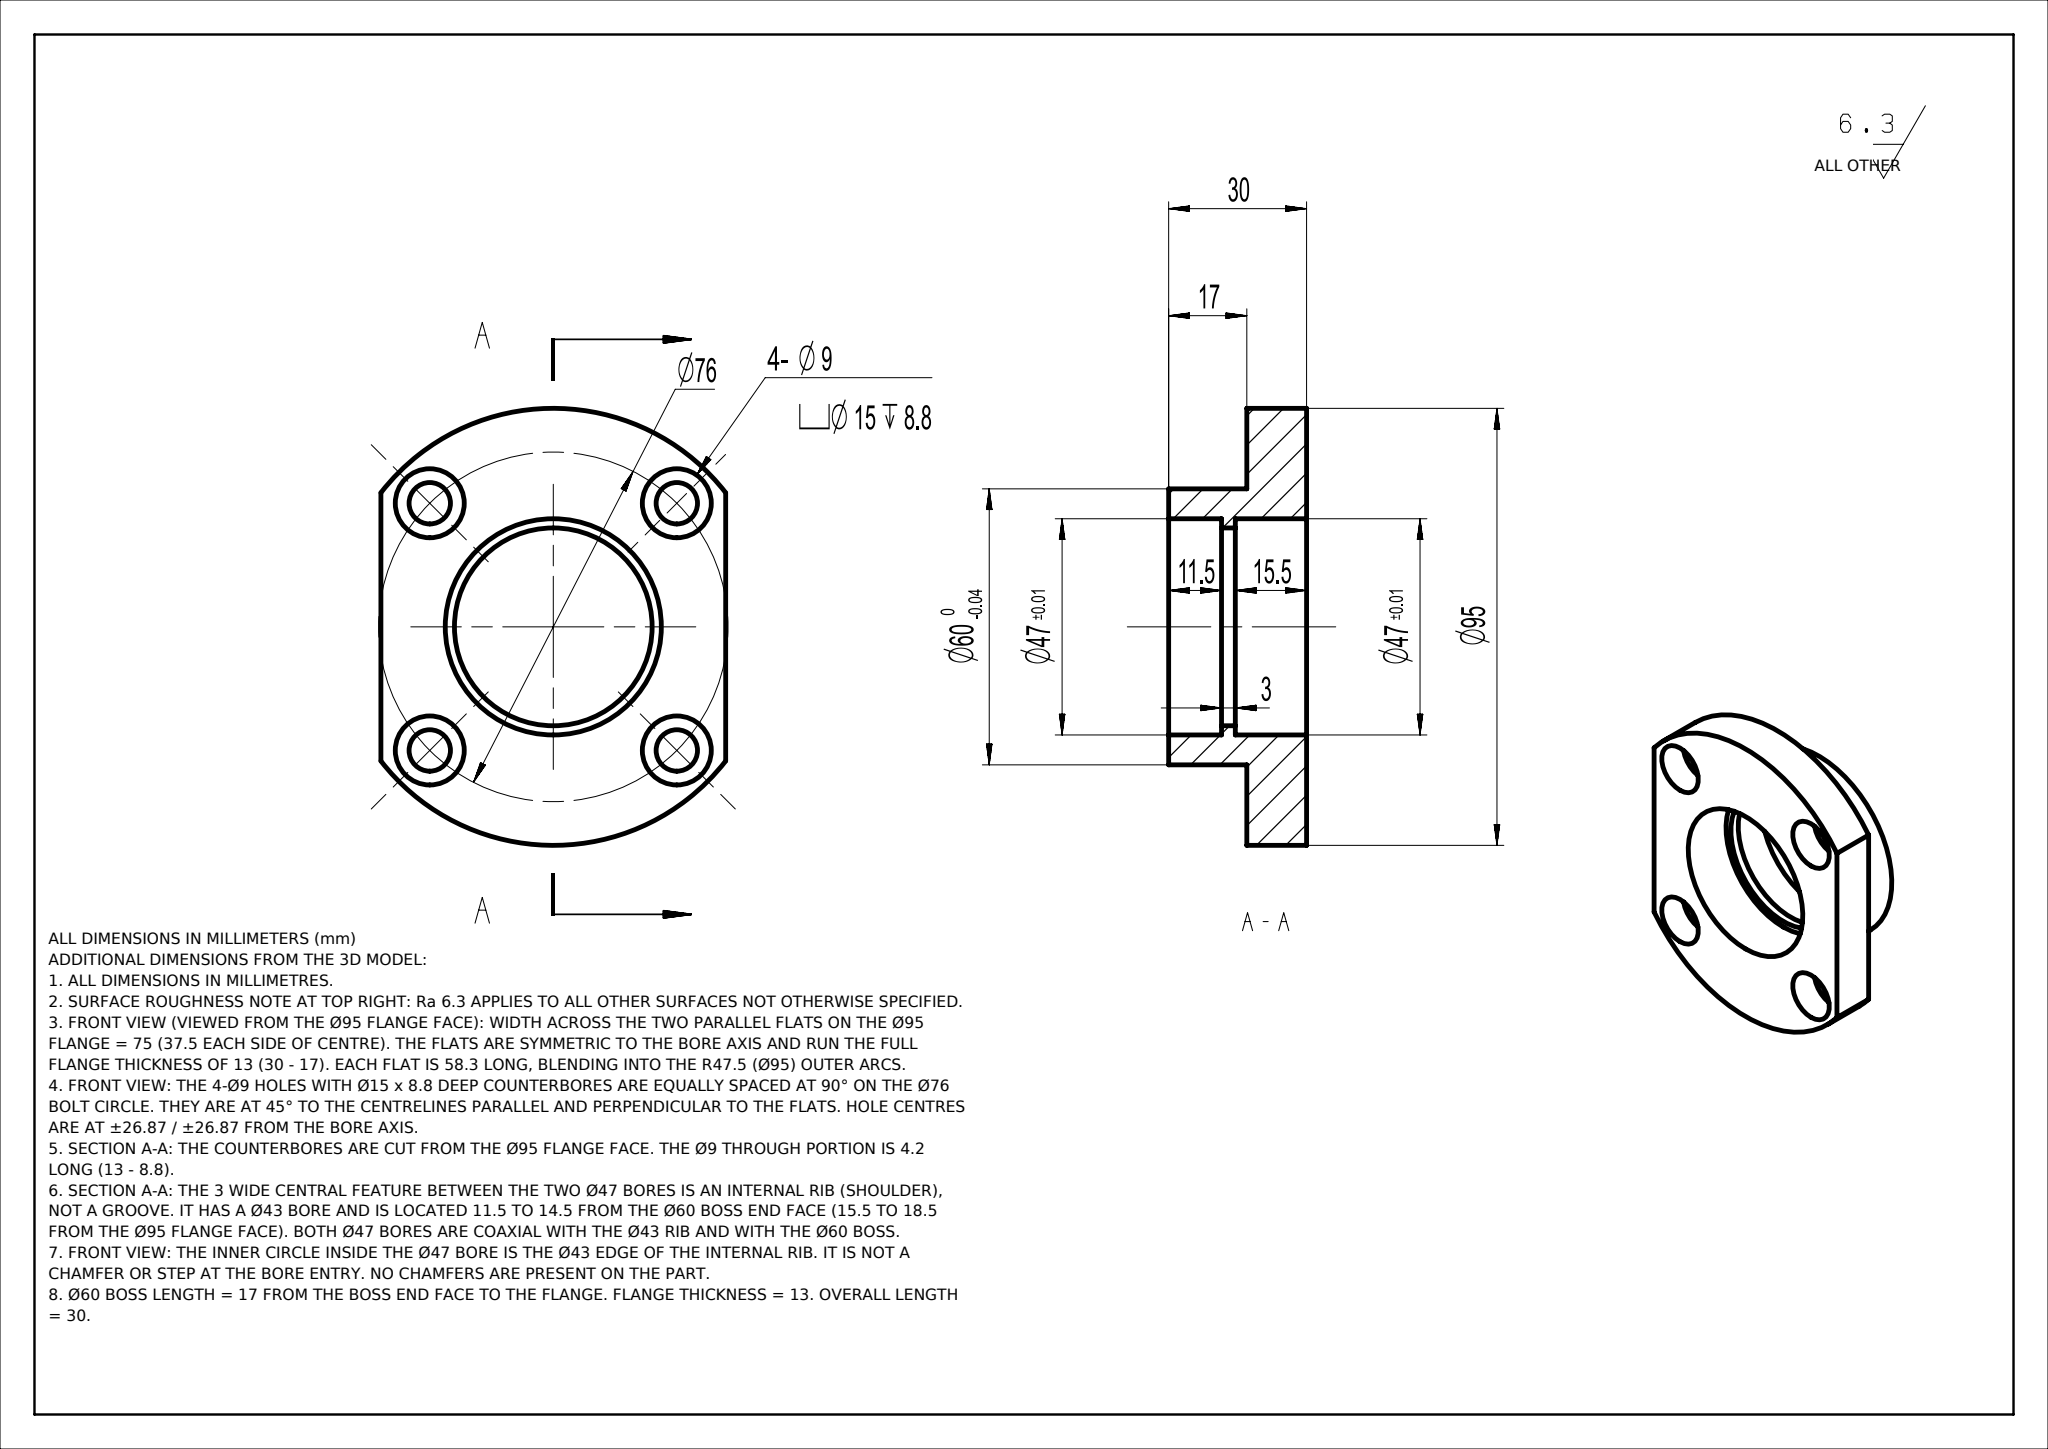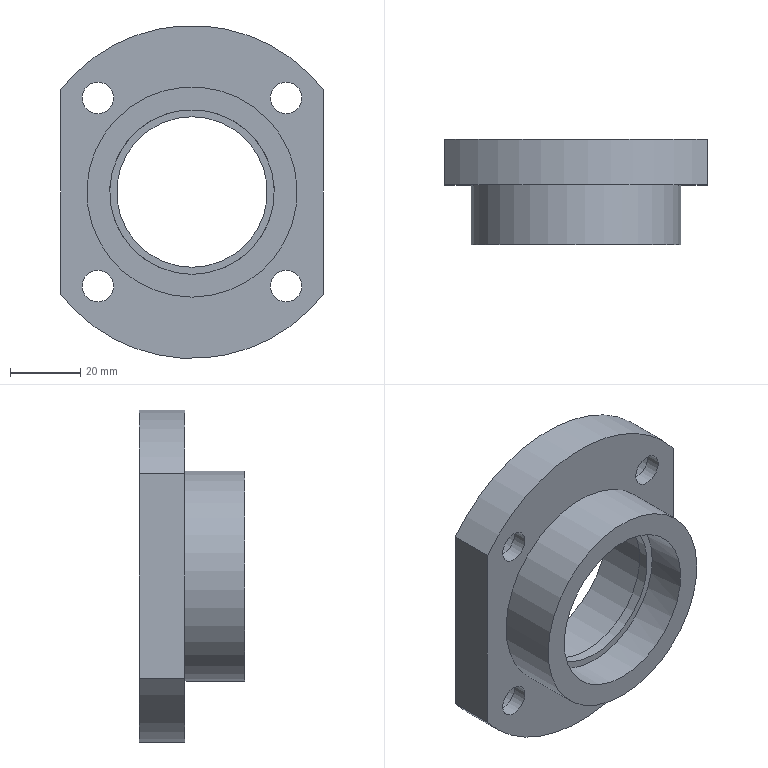Part | NX | mm | 1 solid | 25 faces | box 75 x 30 x 95 mm | volume 71383 mm3 | cylinder 14 | plane 11 | commonest cylinder face diameters 9 x4 15 x4 95 x2 47 x2 60 x1 43 x1
STEP:
#1=CARTESIAN_POINT('',(0.,0.,0.));
#2=DIRECTION('',(0.,0.,1.));
#3=DIRECTION('',(1.,0.,0.));
#4=AXIS2_PLACEMENT_3D('',#1,#2,#3);
#5=(LENGTH_UNIT()NAMED_UNIT(*)SI_UNIT(.MILLI.,.METRE.));
#6=UNCERTAINTY_MEASURE_WITH_UNIT(LENGTH_MEASURE(0.00002),#5,'','');
#7=(NAMED_UNIT(*)PLANE_ANGLE_UNIT()SI_UNIT($,.RADIAN.));
#8=PLANE_ANGLE_MEASURE_WITH_UNIT(PLANE_ANGLE_MEASURE(0.01745),#7);
#9=DIMENSIONAL_EXPONENTS(0.,0.,0.,0.,0.,0.,0.);
#10=(CONVERSION_BASED_UNIT('',#8)NAMED_UNIT(#9)PLANE_ANGLE_UNIT());
#11=(NAMED_UNIT(*)SI_UNIT($,.STERADIAN.)SOLID_ANGLE_UNIT());
#12=(GEOMETRIC_REPRESENTATION_CONTEXT(3)GLOBAL_UNCERTAINTY_ASSIGNED_CONTEXT((#6))GLOBAL_UNIT_ASSIGNED_CONTEXT((#5,#10,#11))REPRESENTATION_CONTEXT('',''));
#13=SHAPE_REPRESENTATION('',(#4),#12);
#14=CARTESIAN_POINT('',(37.5,30.,29.155));
#15=VERTEX_POINT('',#14);
#16=CARTESIAN_POINT('',(-37.5,30.,29.155));
#17=VERTEX_POINT('',#16);
#18=CARTESIAN_POINT('',(0.,30.,0.));
#19=DIRECTION('',(0.,-1.,0.));
#20=DIRECTION('',(0.,0.,-1.));
#21=AXIS2_PLACEMENT_3D('',#18,#19,#20);
#22=CIRCLE('',#21,47.5);
#23=EDGE_CURVE('',#15,#17,#22,.T.);
#24=ORIENTED_EDGE('',*,*,#23,.T.);
#25=CARTESIAN_POINT('',(-37.5,17.,29.155));
#26=VERTEX_POINT('',#25);
#27=CARTESIAN_POINT('',(-37.5,0.,29.155));
#28=DIRECTION('',(0.,-1.,0.));
#29=VECTOR('',#28,1.);
#30=LINE('',#27,#29);
#31=EDGE_CURVE('',#17,#26,#30,.T.);
#32=ORIENTED_EDGE('',*,*,#31,.T.);
#33=CARTESIAN_POINT('',(37.5,17.,29.155));
#34=VERTEX_POINT('',#33);
#35=CARTESIAN_POINT('',(0.,17.,0.));
#36=DIRECTION('',(0.,-1.,0.));
#37=DIRECTION('',(0.,0.,-1.));
#38=AXIS2_PLACEMENT_3D('',#35,#36,#37);
#39=CIRCLE('',#38,47.5);
#40=EDGE_CURVE('',#34,#26,#39,.T.);
#41=ORIENTED_EDGE('',*,*,#40,.F.);
#42=CARTESIAN_POINT('',(37.5,0.,29.155));
#43=DIRECTION('',(0.,1.,0.));
#44=VECTOR('',#43,1.);
#45=LINE('',#42,#44);
#46=EDGE_CURVE('',#34,#15,#45,.T.);
#47=ORIENTED_EDGE('',*,*,#46,.T.);
#48=EDGE_LOOP('',(#24,#32,#41,#47));
#49=FACE_OUTER_BOUND('',#48,.T.);
#50=CARTESIAN_POINT('',(0.,0.,0.));
#51=DIRECTION('',(0.,-1.,0.));
#52=DIRECTION('',(0.,0.,-1.));
#53=AXIS2_PLACEMENT_3D('',#50,#51,#52);
#54=CYLINDRICAL_SURFACE('',#53,47.5);
#55=ADVANCED_FACE('',(#49),#54,.T.);
#56=CARTESIAN_POINT('',(0.,-0.,-23.5));
#57=VERTEX_POINT('',#56);
#58=CARTESIAN_POINT('',(0.,-0.,0.));
#59=DIRECTION('',(0.,-1.,0.));
#60=DIRECTION('',(0.,0.,-1.));
#61=AXIS2_PLACEMENT_3D('',#58,#59,#60);
#62=CIRCLE('',#61,23.5);
#63=EDGE_CURVE('',#57,#57,#62,.T.);
#64=ORIENTED_EDGE('',*,*,#63,.T.);
#65=EDGE_LOOP('',(#64));
#66=FACE_BOUND('',#65,.T.);
#67=CARTESIAN_POINT('',(0.,11.5,23.5));
#68=VERTEX_POINT('',#67);
#69=CARTESIAN_POINT('',(0.,11.5,0.));
#70=DIRECTION('',(0.,-1.,0.));
#71=DIRECTION('',(0.,0.,1.));
#72=AXIS2_PLACEMENT_3D('',#69,#70,#71);
#73=CIRCLE('',#72,23.5);
#74=EDGE_CURVE('',#68,#68,#73,.T.);
#75=ORIENTED_EDGE('',*,*,#74,.F.);
#76=EDGE_LOOP('',(#75));
#77=FACE_BOUND('',#76,.T.);
#78=CARTESIAN_POINT('',(0.,0.,0.));
#79=DIRECTION('',(0.,-1.,0.));
#80=DIRECTION('',(0.,0.,-1.));
#81=AXIS2_PLACEMENT_3D('',#78,#79,#80);
#82=CYLINDRICAL_SURFACE('',#81,23.5);
#83=ADVANCED_FACE('',(#66,#77),#82,.F.);
#84=ORIENTED_EDGE('',*,*,#63,.F.);
#85=EDGE_LOOP('',(#84));
#86=FACE_BOUND('',#85,.T.);
#87=CARTESIAN_POINT('',(0.,-0.,-30.));
#88=VERTEX_POINT('',#87);
#89=CARTESIAN_POINT('',(0.,-0.,0.));
#90=DIRECTION('',(0.,-1.,0.));
#91=DIRECTION('',(0.,0.,-1.));
#92=AXIS2_PLACEMENT_3D('',#89,#90,#91);
#93=CIRCLE('',#92,30.);
#94=EDGE_CURVE('',#88,#88,#93,.T.);
#95=ORIENTED_EDGE('',*,*,#94,.T.);
#96=EDGE_LOOP('',(#95));
#97=FACE_BOUND('',#96,.T.);
#98=CARTESIAN_POINT('',(0.,-0.,30.));
#99=DIRECTION('',(0.,1.,0.));
#100=DIRECTION('',(0.,0.,1.));
#101=AXIS2_PLACEMENT_3D('',#98,#99,#100);
#102=PLANE('',#101);
#103=ADVANCED_FACE('',(#86,#97),#102,.F.);
#104=CARTESIAN_POINT('',(0.,14.5,-23.5));
#105=VERTEX_POINT('',#104);
#106=CARTESIAN_POINT('',(0.,14.5,0.));
#107=DIRECTION('',(0.,-1.,0.));
#108=DIRECTION('',(0.,0.,-1.));
#109=AXIS2_PLACEMENT_3D('',#106,#107,#108);
#110=CIRCLE('',#109,23.5);
#111=EDGE_CURVE('',#105,#105,#110,.T.);
#112=ORIENTED_EDGE('',*,*,#111,.T.);
#113=EDGE_LOOP('',(#112));
#114=FACE_BOUND('',#113,.T.);
#115=CARTESIAN_POINT('',(0.,30.,-23.5));
#116=VERTEX_POINT('',#115);
#117=CARTESIAN_POINT('',(0.,30.,0.));
#118=DIRECTION('',(0.,-1.,0.));
#119=DIRECTION('',(0.,0.,-1.));
#120=AXIS2_PLACEMENT_3D('',#117,#118,#119);
#121=CIRCLE('',#120,23.5);
#122=EDGE_CURVE('',#116,#116,#121,.T.);
#123=ORIENTED_EDGE('',*,*,#122,.F.);
#124=EDGE_LOOP('',(#123));
#125=FACE_BOUND('',#124,.T.);
#126=CARTESIAN_POINT('',(0.,0.,0.));
#127=DIRECTION('',(0.,-1.,0.));
#128=DIRECTION('',(0.,0.,-1.));
#129=AXIS2_PLACEMENT_3D('',#126,#127,#128);
#130=CYLINDRICAL_SURFACE('',#129,23.5);
#131=ADVANCED_FACE('',(#114,#125),#130,.F.);
#132=CARTESIAN_POINT('',(26.87,30.,19.37));
#133=VERTEX_POINT('',#132);
#134=CARTESIAN_POINT('',(26.87,30.,26.87));
#135=DIRECTION('',(0.,-1.,0.));
#136=DIRECTION('',(0.,0.,-1.));
#137=AXIS2_PLACEMENT_3D('',#134,#135,#136);
#138=CIRCLE('',#137,7.5);
#139=EDGE_CURVE('',#133,#133,#138,.T.);
#140=ORIENTED_EDGE('',*,*,#139,.T.);
#141=EDGE_LOOP('',(#140));
#142=FACE_BOUND('',#141,.T.);
#143=CARTESIAN_POINT('',(26.87,30.,-34.37));
#144=VERTEX_POINT('',#143);
#145=CARTESIAN_POINT('',(26.87,30.,-26.87));
#146=DIRECTION('',(0.,-1.,0.));
#147=DIRECTION('',(0.,0.,-1.));
#148=AXIS2_PLACEMENT_3D('',#145,#146,#147);
#149=CIRCLE('',#148,7.5);
#150=EDGE_CURVE('',#144,#144,#149,.T.);
#151=ORIENTED_EDGE('',*,*,#150,.T.);
#152=EDGE_LOOP('',(#151));
#153=FACE_BOUND('',#152,.T.);
#154=CARTESIAN_POINT('',(-26.87,30.,19.37));
#155=VERTEX_POINT('',#154);
#156=CARTESIAN_POINT('',(-26.87,30.,26.87));
#157=DIRECTION('',(0.,-1.,0.));
#158=DIRECTION('',(0.,0.,-1.));
#159=AXIS2_PLACEMENT_3D('',#156,#157,#158);
#160=CIRCLE('',#159,7.5);
#161=EDGE_CURVE('',#155,#155,#160,.T.);
#162=ORIENTED_EDGE('',*,*,#161,.T.);
#163=EDGE_LOOP('',(#162));
#164=FACE_BOUND('',#163,.T.);
#165=CARTESIAN_POINT('',(-26.87,30.,-34.37));
#166=VERTEX_POINT('',#165);
#167=CARTESIAN_POINT('',(-26.87,30.,-26.87));
#168=DIRECTION('',(0.,-1.,0.));
#169=DIRECTION('',(0.,0.,-1.));
#170=AXIS2_PLACEMENT_3D('',#167,#168,#169);
#171=CIRCLE('',#170,7.5);
#172=EDGE_CURVE('',#166,#166,#171,.T.);
#173=ORIENTED_EDGE('',*,*,#172,.T.);
#174=EDGE_LOOP('',(#173));
#175=FACE_BOUND('',#174,.T.);
#176=ORIENTED_EDGE('',*,*,#23,.F.);
#177=CARTESIAN_POINT('',(37.5,30.,-29.155));
#178=VERTEX_POINT('',#177);
#179=CARTESIAN_POINT('',(37.5,30.,67.008));
#180=DIRECTION('',(0.,0.,-1.));
#181=VECTOR('',#180,1.);
#182=LINE('',#179,#181);
#183=EDGE_CURVE('',#15,#178,#182,.T.);
#184=ORIENTED_EDGE('',*,*,#183,.T.);
#185=CARTESIAN_POINT('',(-37.5,30.,-29.155));
#186=VERTEX_POINT('',#185);
#187=CARTESIAN_POINT('',(0.,30.,0.));
#188=DIRECTION('',(0.,-1.,0.));
#189=DIRECTION('',(0.,0.,-1.));
#190=AXIS2_PLACEMENT_3D('',#187,#188,#189);
#191=CIRCLE('',#190,47.5);
#192=EDGE_CURVE('',#186,#178,#191,.T.);
#193=ORIENTED_EDGE('',*,*,#192,.F.);
#194=CARTESIAN_POINT('',(-37.5,30.,-58.992));
#195=DIRECTION('',(0.,0.,1.));
#196=VECTOR('',#195,1.);
#197=LINE('',#194,#196);
#198=EDGE_CURVE('',#186,#17,#197,.T.);
#199=ORIENTED_EDGE('',*,*,#198,.T.);
#200=EDGE_LOOP('',(#176,#184,#193,#199));
#201=FACE_BOUND('',#200,.T.);
#202=ORIENTED_EDGE('',*,*,#122,.T.);
#203=EDGE_LOOP('',(#202));
#204=FACE_BOUND('',#203,.T.);
#205=CARTESIAN_POINT('',(0.,30.,23.5));
#206=DIRECTION('',(0.,-1.,0.));
#207=DIRECTION('',(0.,0.,-1.));
#208=AXIS2_PLACEMENT_3D('',#205,#206,#207);
#209=PLANE('',#208);
#210=ADVANCED_FACE('',(#142,#153,#164,#175,#201,#204),#209,.F.);
#211=CARTESIAN_POINT('',(-37.5,17.,-29.155));
#212=VERTEX_POINT('',#211);
#213=CARTESIAN_POINT('',(37.5,17.,-29.155));
#214=VERTEX_POINT('',#213);
#215=CARTESIAN_POINT('',(0.,17.,0.));
#216=DIRECTION('',(0.,-1.,0.));
#217=DIRECTION('',(0.,0.,-1.));
#218=AXIS2_PLACEMENT_3D('',#215,#216,#217);
#219=CIRCLE('',#218,47.5);
#220=EDGE_CURVE('',#212,#214,#219,.T.);
#221=ORIENTED_EDGE('',*,*,#220,.F.);
#222=CARTESIAN_POINT('',(-37.5,0.,-29.155));
#223=DIRECTION('',(0.,1.,0.));
#224=VECTOR('',#223,1.);
#225=LINE('',#222,#224);
#226=EDGE_CURVE('',#212,#186,#225,.T.);
#227=ORIENTED_EDGE('',*,*,#226,.T.);
#228=ORIENTED_EDGE('',*,*,#192,.T.);
#229=CARTESIAN_POINT('',(37.5,0.,-29.155));
#230=DIRECTION('',(0.,-1.,0.));
#231=VECTOR('',#230,1.);
#232=LINE('',#229,#231);
#233=EDGE_CURVE('',#178,#214,#232,.T.);
#234=ORIENTED_EDGE('',*,*,#233,.T.);
#235=EDGE_LOOP('',(#221,#227,#228,#234));
#236=FACE_OUTER_BOUND('',#235,.T.);
#237=CARTESIAN_POINT('',(0.,0.,0.));
#238=DIRECTION('',(0.,-1.,0.));
#239=DIRECTION('',(0.,0.,-1.));
#240=AXIS2_PLACEMENT_3D('',#237,#238,#239);
#241=CYLINDRICAL_SURFACE('',#240,47.5);
#242=ADVANCED_FACE('',(#236),#241,.T.);
#243=CARTESIAN_POINT('',(26.87,17.,31.37));
#244=VERTEX_POINT('',#243);
#245=CARTESIAN_POINT('',(26.87,17.,26.87));
#246=DIRECTION('',(0.,1.,0.));
#247=DIRECTION('',(0.,0.,1.));
#248=AXIS2_PLACEMENT_3D('',#245,#246,#247);
#249=CIRCLE('',#248,4.5);
#250=EDGE_CURVE('',#244,#244,#249,.T.);
#251=ORIENTED_EDGE('',*,*,#250,.T.);
#252=EDGE_LOOP('',(#251));
#253=FACE_BOUND('',#252,.T.);
#254=CARTESIAN_POINT('',(26.87,17.,-22.37));
#255=VERTEX_POINT('',#254);
#256=CARTESIAN_POINT('',(26.87,17.,-26.87));
#257=DIRECTION('',(0.,1.,0.));
#258=DIRECTION('',(0.,0.,1.));
#259=AXIS2_PLACEMENT_3D('',#256,#257,#258);
#260=CIRCLE('',#259,4.5);
#261=EDGE_CURVE('',#255,#255,#260,.T.);
#262=ORIENTED_EDGE('',*,*,#261,.T.);
#263=EDGE_LOOP('',(#262));
#264=FACE_BOUND('',#263,.T.);
#265=CARTESIAN_POINT('',(-26.87,17.,31.37));
#266=VERTEX_POINT('',#265);
#267=CARTESIAN_POINT('',(-26.87,17.,26.87));
#268=DIRECTION('',(0.,1.,0.));
#269=DIRECTION('',(0.,0.,1.));
#270=AXIS2_PLACEMENT_3D('',#267,#268,#269);
#271=CIRCLE('',#270,4.5);
#272=EDGE_CURVE('',#266,#266,#271,.T.);
#273=ORIENTED_EDGE('',*,*,#272,.T.);
#274=EDGE_LOOP('',(#273));
#275=FACE_BOUND('',#274,.T.);
#276=CARTESIAN_POINT('',(-26.87,17.,-22.37));
#277=VERTEX_POINT('',#276);
#278=CARTESIAN_POINT('',(-26.87,17.,-26.87));
#279=DIRECTION('',(0.,1.,0.));
#280=DIRECTION('',(0.,0.,1.));
#281=AXIS2_PLACEMENT_3D('',#278,#279,#280);
#282=CIRCLE('',#281,4.5);
#283=EDGE_CURVE('',#277,#277,#282,.T.);
#284=ORIENTED_EDGE('',*,*,#283,.T.);
#285=EDGE_LOOP('',(#284));
#286=FACE_BOUND('',#285,.T.);
#287=CARTESIAN_POINT('',(0.,17.,-30.));
#288=VERTEX_POINT('',#287);
#289=CARTESIAN_POINT('',(0.,17.,0.));
#290=DIRECTION('',(0.,-1.,0.));
#291=DIRECTION('',(0.,0.,-1.));
#292=AXIS2_PLACEMENT_3D('',#289,#290,#291);
#293=CIRCLE('',#292,30.);
#294=EDGE_CURVE('',#288,#288,#293,.T.);
#295=ORIENTED_EDGE('',*,*,#294,.F.);
#296=EDGE_LOOP('',(#295));
#297=FACE_BOUND('',#296,.T.);
#298=ORIENTED_EDGE('',*,*,#40,.T.);
#299=CARTESIAN_POINT('',(-37.5,17.,47.5));
#300=DIRECTION('',(-0.,0.,-1.));
#301=VECTOR('',#300,1.);
#302=LINE('',#299,#301);
#303=EDGE_CURVE('',#26,#212,#302,.T.);
#304=ORIENTED_EDGE('',*,*,#303,.T.);
#305=ORIENTED_EDGE('',*,*,#220,.T.);
#306=CARTESIAN_POINT('',(37.5,17.,47.5));
#307=DIRECTION('',(-0.,0.,1.));
#308=VECTOR('',#307,1.);
#309=LINE('',#306,#308);
#310=EDGE_CURVE('',#214,#34,#309,.T.);
#311=ORIENTED_EDGE('',*,*,#310,.T.);
#312=EDGE_LOOP('',(#298,#304,#305,#311));
#313=FACE_BOUND('',#312,.T.);
#314=CARTESIAN_POINT('',(0.,17.,47.5));
#315=DIRECTION('',(0.,1.,0.));
#316=DIRECTION('',(0.,0.,1.));
#317=AXIS2_PLACEMENT_3D('',#314,#315,#316);
#318=PLANE('',#317);
#319=ADVANCED_FACE('',(#253,#264,#275,#286,#297,#313),#318,.F.);
#320=ORIENTED_EDGE('',*,*,#94,.F.);
#321=EDGE_LOOP('',(#320));
#322=FACE_BOUND('',#321,.T.);
#323=ORIENTED_EDGE('',*,*,#294,.T.);
#324=EDGE_LOOP('',(#323));
#325=FACE_BOUND('',#324,.T.);
#326=CARTESIAN_POINT('',(0.,0.,0.));
#327=DIRECTION('',(0.,-1.,0.));
#328=DIRECTION('',(0.,0.,-1.));
#329=AXIS2_PLACEMENT_3D('',#326,#327,#328);
#330=CYLINDRICAL_SURFACE('',#329,30.);
#331=ADVANCED_FACE('',(#322,#325),#330,.T.);
#332=CARTESIAN_POINT('',(-26.87,21.2,-31.37));
#333=VERTEX_POINT('',#332);
#334=CARTESIAN_POINT('',(-26.87,21.2,-26.87));
#335=DIRECTION('',(0.,1.,0.));
#336=DIRECTION('',(0.,0.,-1.));
#337=AXIS2_PLACEMENT_3D('',#334,#335,#336);
#338=CIRCLE('',#337,4.5);
#339=EDGE_CURVE('',#333,#333,#338,.T.);
#340=ORIENTED_EDGE('',*,*,#339,.T.);
#341=EDGE_LOOP('',(#340));
#342=FACE_BOUND('',#341,.T.);
#343=ORIENTED_EDGE('',*,*,#283,.F.);
#344=EDGE_LOOP('',(#343));
#345=FACE_BOUND('',#344,.T.);
#346=CARTESIAN_POINT('',(-26.87,-10.,-26.87));
#347=DIRECTION('',(0.,-1.,0.));
#348=DIRECTION('',(0.,0.,-1.));
#349=AXIS2_PLACEMENT_3D('',#346,#347,#348);
#350=CYLINDRICAL_SURFACE('',#349,4.5);
#351=ADVANCED_FACE('',(#342,#345),#350,.F.);
#352=ORIENTED_EDGE('',*,*,#339,.F.);
#353=EDGE_LOOP('',(#352));
#354=FACE_BOUND('',#353,.T.);
#355=CARTESIAN_POINT('',(-26.87,21.2,-34.37));
#356=VERTEX_POINT('',#355);
#357=CARTESIAN_POINT('',(-26.87,21.2,-26.87));
#358=DIRECTION('',(0.,1.,0.));
#359=DIRECTION('',(0.,0.,-1.));
#360=AXIS2_PLACEMENT_3D('',#357,#358,#359);
#361=CIRCLE('',#360,7.5);
#362=EDGE_CURVE('',#356,#356,#361,.T.);
#363=ORIENTED_EDGE('',*,*,#362,.T.);
#364=EDGE_LOOP('',(#363));
#365=FACE_BOUND('',#364,.T.);
#366=CARTESIAN_POINT('',(-26.87,21.2,-26.87));
#367=DIRECTION('',(0.,-1.,0.));
#368=DIRECTION('',(0.,0.,-1.));
#369=AXIS2_PLACEMENT_3D('',#366,#367,#368);
#370=PLANE('',#369);
#371=ADVANCED_FACE('',(#354,#365),#370,.F.);
#372=ORIENTED_EDGE('',*,*,#362,.F.);
#373=EDGE_LOOP('',(#372));
#374=FACE_BOUND('',#373,.T.);
#375=ORIENTED_EDGE('',*,*,#172,.F.);
#376=EDGE_LOOP('',(#375));
#377=FACE_BOUND('',#376,.T.);
#378=CARTESIAN_POINT('',(-26.87,30.,-26.87));
#379=DIRECTION('',(0.,-1.,0.));
#380=DIRECTION('',(0.,0.,-1.));
#381=AXIS2_PLACEMENT_3D('',#378,#379,#380);
#382=CYLINDRICAL_SURFACE('',#381,7.5);
#383=ADVANCED_FACE('',(#374,#377),#382,.F.);
#384=CARTESIAN_POINT('',(-26.87,21.2,22.37));
#385=VERTEX_POINT('',#384);
#386=CARTESIAN_POINT('',(-26.87,21.2,26.87));
#387=DIRECTION('',(0.,1.,0.));
#388=DIRECTION('',(0.,0.,-1.));
#389=AXIS2_PLACEMENT_3D('',#386,#387,#388);
#390=CIRCLE('',#389,4.5);
#391=EDGE_CURVE('',#385,#385,#390,.T.);
#392=ORIENTED_EDGE('',*,*,#391,.T.);
#393=EDGE_LOOP('',(#392));
#394=FACE_BOUND('',#393,.T.);
#395=ORIENTED_EDGE('',*,*,#272,.F.);
#396=EDGE_LOOP('',(#395));
#397=FACE_BOUND('',#396,.T.);
#398=CARTESIAN_POINT('',(-26.87,-10.,26.87));
#399=DIRECTION('',(0.,-1.,0.));
#400=DIRECTION('',(0.,0.,-1.));
#401=AXIS2_PLACEMENT_3D('',#398,#399,#400);
#402=CYLINDRICAL_SURFACE('',#401,4.5);
#403=ADVANCED_FACE('',(#394,#397),#402,.F.);
#404=ORIENTED_EDGE('',*,*,#391,.F.);
#405=EDGE_LOOP('',(#404));
#406=FACE_BOUND('',#405,.T.);
#407=CARTESIAN_POINT('',(-26.87,21.2,19.37));
#408=VERTEX_POINT('',#407);
#409=CARTESIAN_POINT('',(-26.87,21.2,26.87));
#410=DIRECTION('',(0.,1.,0.));
#411=DIRECTION('',(0.,0.,-1.));
#412=AXIS2_PLACEMENT_3D('',#409,#410,#411);
#413=CIRCLE('',#412,7.5);
#414=EDGE_CURVE('',#408,#408,#413,.T.);
#415=ORIENTED_EDGE('',*,*,#414,.T.);
#416=EDGE_LOOP('',(#415));
#417=FACE_BOUND('',#416,.T.);
#418=CARTESIAN_POINT('',(-26.87,21.2,26.87));
#419=DIRECTION('',(0.,-1.,0.));
#420=DIRECTION('',(0.,0.,-1.));
#421=AXIS2_PLACEMENT_3D('',#418,#419,#420);
#422=PLANE('',#421);
#423=ADVANCED_FACE('',(#406,#417),#422,.F.);
#424=ORIENTED_EDGE('',*,*,#414,.F.);
#425=EDGE_LOOP('',(#424));
#426=FACE_BOUND('',#425,.T.);
#427=ORIENTED_EDGE('',*,*,#161,.F.);
#428=EDGE_LOOP('',(#427));
#429=FACE_BOUND('',#428,.T.);
#430=CARTESIAN_POINT('',(-26.87,30.,26.87));
#431=DIRECTION('',(0.,-1.,0.));
#432=DIRECTION('',(0.,0.,-1.));
#433=AXIS2_PLACEMENT_3D('',#430,#431,#432);
#434=CYLINDRICAL_SURFACE('',#433,7.5);
#435=ADVANCED_FACE('',(#426,#429),#434,.F.);
#436=CARTESIAN_POINT('',(26.87,21.2,-31.37));
#437=VERTEX_POINT('',#436);
#438=CARTESIAN_POINT('',(26.87,21.2,-26.87));
#439=DIRECTION('',(0.,1.,0.));
#440=DIRECTION('',(0.,0.,-1.));
#441=AXIS2_PLACEMENT_3D('',#438,#439,#440);
#442=CIRCLE('',#441,4.5);
#443=EDGE_CURVE('',#437,#437,#442,.T.);
#444=ORIENTED_EDGE('',*,*,#443,.T.);
#445=EDGE_LOOP('',(#444));
#446=FACE_BOUND('',#445,.T.);
#447=ORIENTED_EDGE('',*,*,#261,.F.);
#448=EDGE_LOOP('',(#447));
#449=FACE_BOUND('',#448,.T.);
#450=CARTESIAN_POINT('',(26.87,-10.,-26.87));
#451=DIRECTION('',(0.,-1.,0.));
#452=DIRECTION('',(0.,0.,-1.));
#453=AXIS2_PLACEMENT_3D('',#450,#451,#452);
#454=CYLINDRICAL_SURFACE('',#453,4.5);
#455=ADVANCED_FACE('',(#446,#449),#454,.F.);
#456=ORIENTED_EDGE('',*,*,#443,.F.);
#457=EDGE_LOOP('',(#456));
#458=FACE_BOUND('',#457,.T.);
#459=CARTESIAN_POINT('',(26.87,21.2,-34.37));
#460=VERTEX_POINT('',#459);
#461=CARTESIAN_POINT('',(26.87,21.2,-26.87));
#462=DIRECTION('',(0.,1.,0.));
#463=DIRECTION('',(0.,0.,-1.));
#464=AXIS2_PLACEMENT_3D('',#461,#462,#463);
#465=CIRCLE('',#464,7.5);
#466=EDGE_CURVE('',#460,#460,#465,.T.);
#467=ORIENTED_EDGE('',*,*,#466,.T.);
#468=EDGE_LOOP('',(#467));
#469=FACE_BOUND('',#468,.T.);
#470=CARTESIAN_POINT('',(26.87,21.2,-26.87));
#471=DIRECTION('',(0.,-1.,0.));
#472=DIRECTION('',(0.,0.,-1.));
#473=AXIS2_PLACEMENT_3D('',#470,#471,#472);
#474=PLANE('',#473);
#475=ADVANCED_FACE('',(#458,#469),#474,.F.);
#476=ORIENTED_EDGE('',*,*,#466,.F.);
#477=EDGE_LOOP('',(#476));
#478=FACE_BOUND('',#477,.T.);
#479=ORIENTED_EDGE('',*,*,#150,.F.);
#480=EDGE_LOOP('',(#479));
#481=FACE_BOUND('',#480,.T.);
#482=CARTESIAN_POINT('',(26.87,30.,-26.87));
#483=DIRECTION('',(0.,-1.,0.));
#484=DIRECTION('',(0.,0.,-1.));
#485=AXIS2_PLACEMENT_3D('',#482,#483,#484);
#486=CYLINDRICAL_SURFACE('',#485,7.5);
#487=ADVANCED_FACE('',(#478,#481),#486,.F.);
#488=CARTESIAN_POINT('',(26.87,21.2,22.37));
#489=VERTEX_POINT('',#488);
#490=CARTESIAN_POINT('',(26.87,21.2,26.87));
#491=DIRECTION('',(0.,1.,0.));
#492=DIRECTION('',(0.,0.,-1.));
#493=AXIS2_PLACEMENT_3D('',#490,#491,#492);
#494=CIRCLE('',#493,4.5);
#495=EDGE_CURVE('',#489,#489,#494,.T.);
#496=ORIENTED_EDGE('',*,*,#495,.T.);
#497=EDGE_LOOP('',(#496));
#498=FACE_BOUND('',#497,.T.);
#499=ORIENTED_EDGE('',*,*,#250,.F.);
#500=EDGE_LOOP('',(#499));
#501=FACE_BOUND('',#500,.T.);
#502=CARTESIAN_POINT('',(26.87,-10.,26.87));
#503=DIRECTION('',(0.,-1.,0.));
#504=DIRECTION('',(0.,0.,-1.));
#505=AXIS2_PLACEMENT_3D('',#502,#503,#504);
#506=CYLINDRICAL_SURFACE('',#505,4.5);
#507=ADVANCED_FACE('',(#498,#501),#506,.F.);
#508=ORIENTED_EDGE('',*,*,#495,.F.);
#509=EDGE_LOOP('',(#508));
#510=FACE_BOUND('',#509,.T.);
#511=CARTESIAN_POINT('',(26.87,21.2,19.37));
#512=VERTEX_POINT('',#511);
#513=CARTESIAN_POINT('',(26.87,21.2,26.87));
#514=DIRECTION('',(0.,1.,0.));
#515=DIRECTION('',(0.,0.,-1.));
#516=AXIS2_PLACEMENT_3D('',#513,#514,#515);
#517=CIRCLE('',#516,7.5);
#518=EDGE_CURVE('',#512,#512,#517,.T.);
#519=ORIENTED_EDGE('',*,*,#518,.T.);
#520=EDGE_LOOP('',(#519));
#521=FACE_BOUND('',#520,.T.);
#522=CARTESIAN_POINT('',(26.87,21.2,26.87));
#523=DIRECTION('',(0.,-1.,0.));
#524=DIRECTION('',(0.,0.,-1.));
#525=AXIS2_PLACEMENT_3D('',#522,#523,#524);
#526=PLANE('',#525);
#527=ADVANCED_FACE('',(#510,#521),#526,.F.);
#528=ORIENTED_EDGE('',*,*,#518,.F.);
#529=EDGE_LOOP('',(#528));
#530=FACE_BOUND('',#529,.T.);
#531=ORIENTED_EDGE('',*,*,#139,.F.);
#532=EDGE_LOOP('',(#531));
#533=FACE_BOUND('',#532,.T.);
#534=CARTESIAN_POINT('',(26.87,30.,26.87));
#535=DIRECTION('',(0.,-1.,0.));
#536=DIRECTION('',(0.,0.,-1.));
#537=AXIS2_PLACEMENT_3D('',#534,#535,#536);
#538=CYLINDRICAL_SURFACE('',#537,7.5);
#539=ADVANCED_FACE('',(#530,#533),#538,.F.);
#540=ORIENTED_EDGE('',*,*,#183,.F.);
#541=ORIENTED_EDGE('',*,*,#46,.F.);
#542=ORIENTED_EDGE('',*,*,#310,.F.);
#543=ORIENTED_EDGE('',*,*,#233,.F.);
#544=EDGE_LOOP('',(#540,#541,#542,#543));
#545=FACE_OUTER_BOUND('',#544,.T.);
#546=CARTESIAN_POINT('',(37.5,30.,67.008));
#547=DIRECTION('',(-1.,0.,-0.));
#548=DIRECTION('',(-0.,0.,1.));
#549=AXIS2_PLACEMENT_3D('',#546,#547,#548);
#550=PLANE('',#549);
#551=ADVANCED_FACE('',(#545),#550,.F.);
#552=ORIENTED_EDGE('',*,*,#198,.F.);
#553=ORIENTED_EDGE('',*,*,#226,.F.);
#554=ORIENTED_EDGE('',*,*,#303,.F.);
#555=ORIENTED_EDGE('',*,*,#31,.F.);
#556=EDGE_LOOP('',(#552,#553,#554,#555));
#557=FACE_OUTER_BOUND('',#556,.T.);
#558=CARTESIAN_POINT('',(-37.5,30.,-58.992));
#559=DIRECTION('',(1.,0.,-0.));
#560=DIRECTION('',(-0.,0.,-1.));
#561=AXIS2_PLACEMENT_3D('',#558,#559,#560);
#562=PLANE('',#561);
#563=ADVANCED_FACE('',(#557),#562,.F.);
#564=CARTESIAN_POINT('',(0.,11.5,21.5));
#565=VERTEX_POINT('',#564);
#566=CARTESIAN_POINT('',(0.,11.5,0.));
#567=DIRECTION('',(0.,1.,0.));
#568=DIRECTION('',(0.,0.,1.));
#569=AXIS2_PLACEMENT_3D('',#566,#567,#568);
#570=CIRCLE('',#569,21.5);
#571=EDGE_CURVE('',#565,#565,#570,.T.);
#572=ORIENTED_EDGE('',*,*,#571,.T.);
#573=EDGE_LOOP('',(#572));
#574=FACE_BOUND('',#573,.T.);
#575=ORIENTED_EDGE('',*,*,#74,.T.);
#576=EDGE_LOOP('',(#575));
#577=FACE_BOUND('',#576,.T.);
#578=CARTESIAN_POINT('',(0.,11.5,0.));
#579=DIRECTION('',(0.,-1.,0.));
#580=DIRECTION('',(0.,0.,-1.));
#581=AXIS2_PLACEMENT_3D('',#578,#579,#580);
#582=PLANE('',#581);
#583=ADVANCED_FACE('',(#574,#577),#582,.T.);
#584=CARTESIAN_POINT('',(0.,14.5,21.5));
#585=VERTEX_POINT('',#584);
#586=CARTESIAN_POINT('',(0.,14.5,0.));
#587=DIRECTION('',(0.,1.,0.));
#588=DIRECTION('',(0.,0.,1.));
#589=AXIS2_PLACEMENT_3D('',#586,#587,#588);
#590=CIRCLE('',#589,21.5);
#591=EDGE_CURVE('',#585,#585,#590,.T.);
#592=ORIENTED_EDGE('',*,*,#591,.F.);
#593=EDGE_LOOP('',(#592));
#594=FACE_BOUND('',#593,.T.);
#595=ORIENTED_EDGE('',*,*,#111,.F.);
#596=EDGE_LOOP('',(#595));
#597=FACE_BOUND('',#596,.T.);
#598=CARTESIAN_POINT('',(0.,14.5,0.));
#599=DIRECTION('',(0.,-1.,0.));
#600=DIRECTION('',(0.,0.,-1.));
#601=AXIS2_PLACEMENT_3D('',#598,#599,#600);
#602=PLANE('',#601);
#603=ADVANCED_FACE('',(#594,#597),#602,.F.);
#604=ORIENTED_EDGE('',*,*,#571,.F.);
#605=EDGE_LOOP('',(#604));
#606=FACE_BOUND('',#605,.T.);
#607=ORIENTED_EDGE('',*,*,#591,.T.);
#608=EDGE_LOOP('',(#607));
#609=FACE_BOUND('',#608,.T.);
#610=CARTESIAN_POINT('',(0.,11.65,0.));
#611=DIRECTION('',(0.,1.,0.));
#612=DIRECTION('',(0.,0.,1.));
#613=AXIS2_PLACEMENT_3D('',#610,#611,#612);
#614=CYLINDRICAL_SURFACE('',#613,21.5);
#615=ADVANCED_FACE('',(#606,#609),#614,.F.);
#616=CLOSED_SHELL('',(#55,#83,#103,#131,#210,#242,#319,#331,#351,#371,#383,#403,#423,#435,#455,#475,#487,#507,#527,#539,#551,#563,#583,#603,#615));
#617=MANIFOLD_SOLID_BREP('',#616);
#618=ADVANCED_BREP_SHAPE_REPRESENTATION('',(#617),#12);
#619=SHAPE_REPRESENTATION_RELATIONSHIP('','',#13,#618);
#620=PRESENTATION_LAYER_ASSIGNMENT('','',(#617));
#621=COLOUR_RGB('',0.4902,0.4902,0.4902);
#622=FILL_AREA_STYLE_COLOUR('',#621);
#623=FILL_AREA_STYLE('',(#622));
#624=SURFACE_STYLE_FILL_AREA(#623);
#625=SURFACE_SIDE_STYLE('',(#624));
#626=SURFACE_STYLE_USAGE(.BOTH.,#625);
#627=PRESENTATION_STYLE_ASSIGNMENT((#626));
#628=STYLED_ITEM('',(#627),#617);
#629=MECHANICAL_DESIGN_GEOMETRIC_PRESENTATION_REPRESENTATION('',(#628),#12);